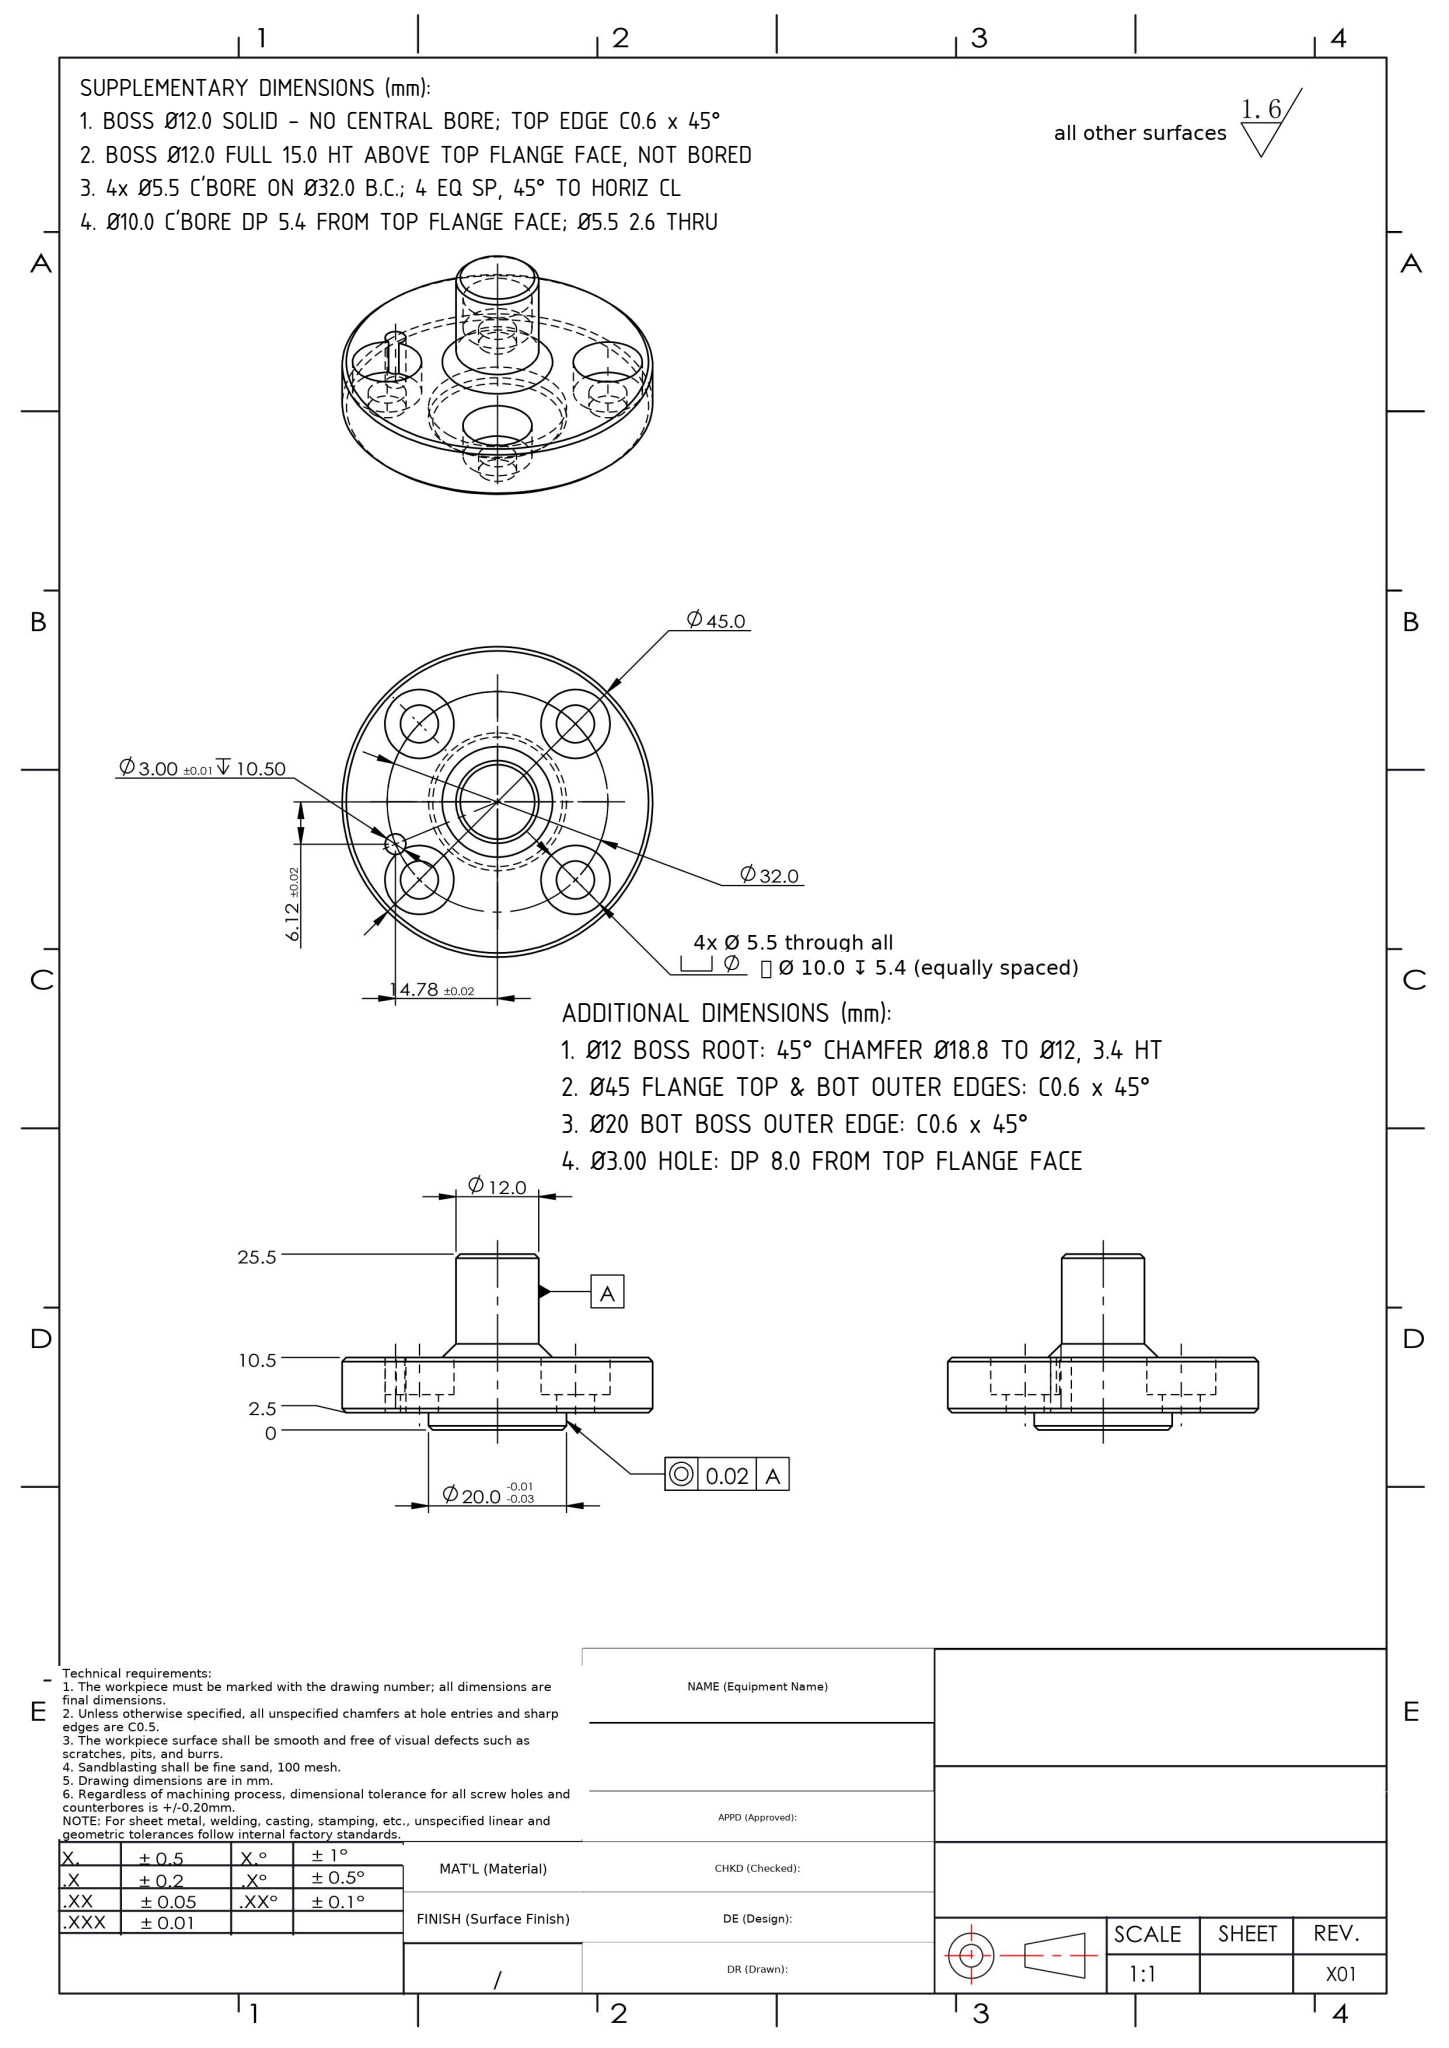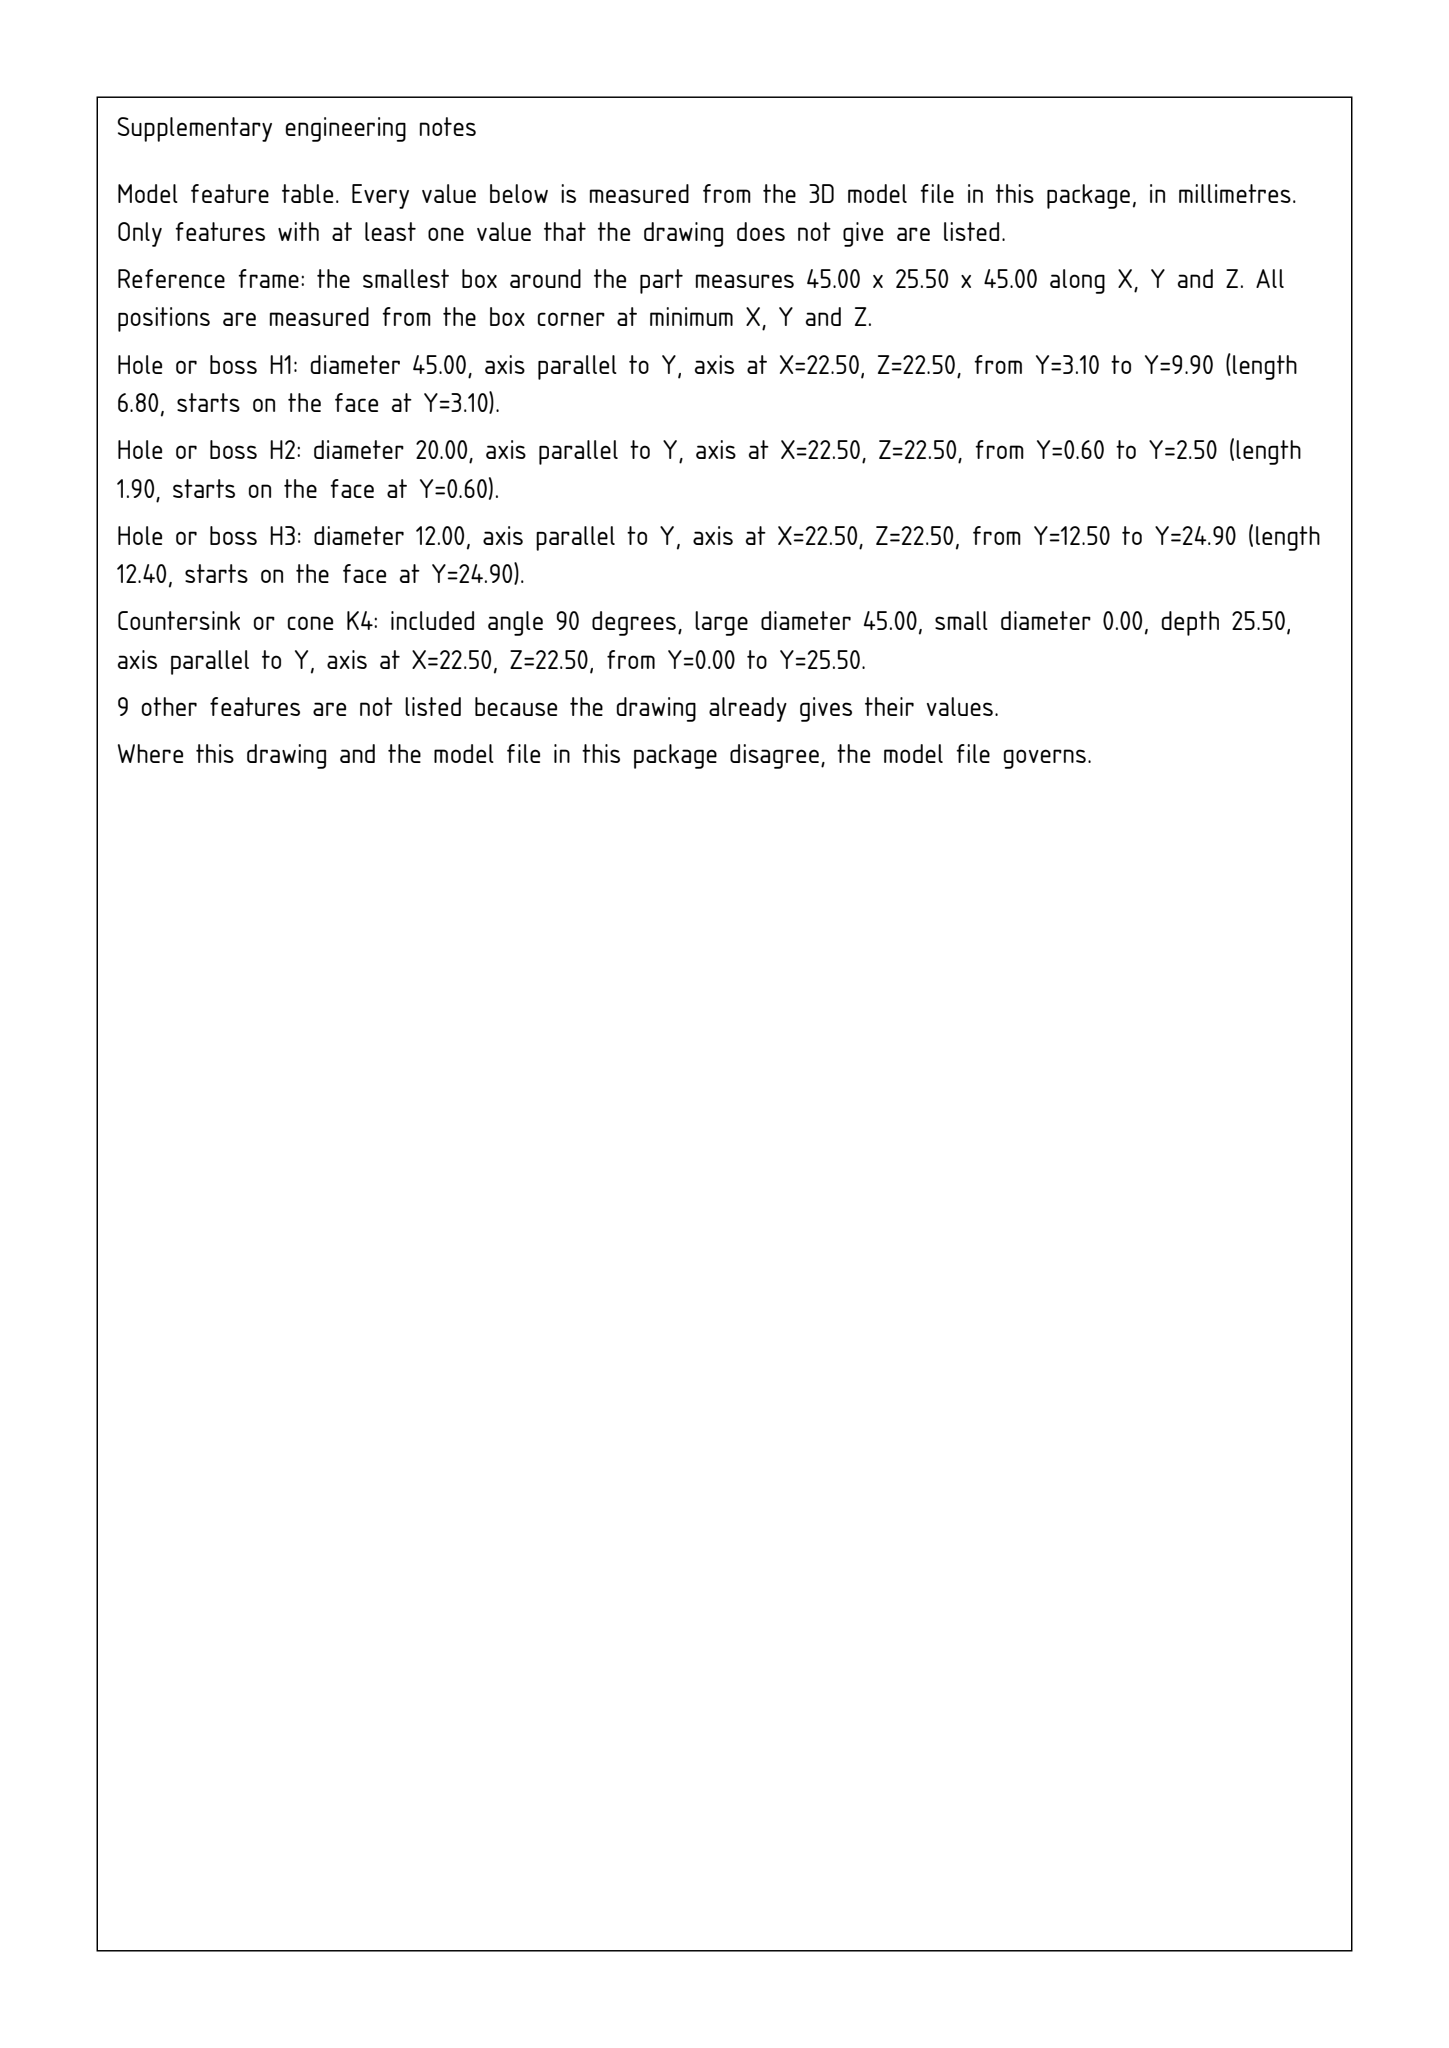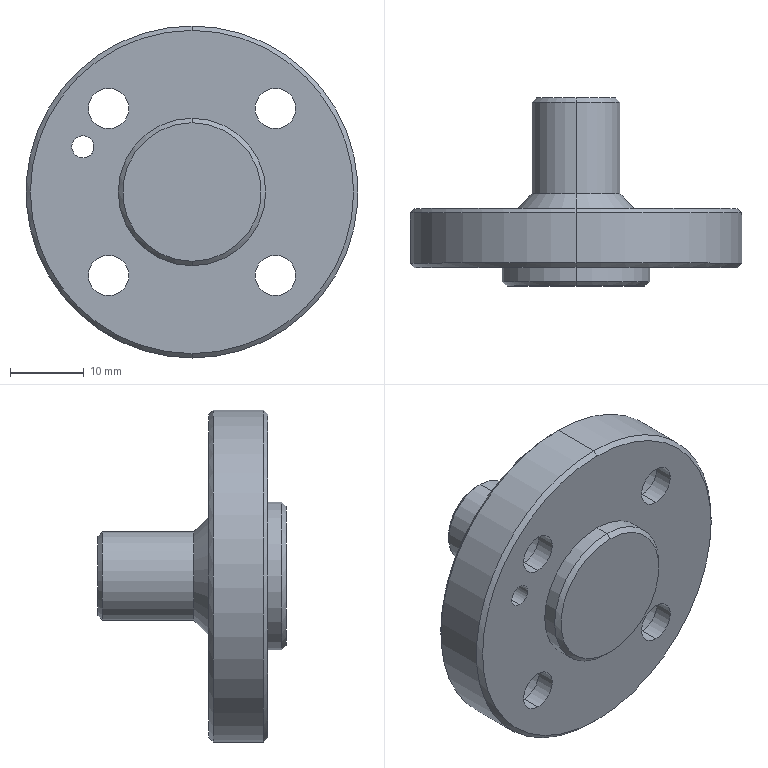Part | SolidWorks | mm | 1 solid | 43 faces | box 45 x 25.5 x 45 mm | volume 13222 mm3 | cylinder 25 | cone 10 | plane 8 | commonest cylinder face diameters 10 x9 5.5 x8 3 x2 20 x2 12 x2 45 x2
build123d program:
from build123d import *

# Parameters (mm, degrees)
SKETCH1_R                                       = 22.5
BOSS_EXTRUDE1_DEPTH                             = 8
SKETCH2_R                                       = 6
BOSS_EXTRUDE2_DEPTH                             = 15
SKETCH3_R                                       = 10
BOSS_EXTRUDE3_DEPTH                             = 2.5
M5_HEX_SOCKET_HEAD_CAP_SCREW_CBORE1_D           = 5.5
M5_HEX_SOCKET_HEAD_CAP_SCREW_CBORE1_CBORE_D     = 10
M5_HEX_SOCKET_HEAD_CAP_SCREW_CBORE1_CBORE_DEPTH = 5.4
CIRPATTERN1_COUNT                               = 4
HOLE1_D                                         = 3
CHAMFER1_SIZE                                   = 0.6
CHAMFER2_SIZE                                   = 2


with BuildPart() as part:
    # Sketch1 → Boss-Extrude1 (new body)
    with BuildSketch(Plane(origin=(0, 0, 0), x_dir=(1, 0, 0), z_dir=(0, 1, 0))):
        with Locations(Location((0, 0, 0), (0, 0, 270))):
            Circle(SKETCH1_R)
    extrude(amount=BOSS_EXTRUDE1_DEPTH)

    # Sketch2 → Boss-Extrude2 (add)
    with BuildSketch(Plane(origin=(0, 8, 0), x_dir=(1, 0, 0), z_dir=(0, 1, 0))):
        with Locations(Location((0, 0, 0), (0, 0, 270))):
            Circle(SKETCH2_R)
    extrude(amount=BOSS_EXTRUDE2_DEPTH)

    # Sketch3 → Boss-Extrude3 (add)
    with BuildSketch(Plane.XZ):
        with Locations(Location((0, 0, 0), (0, 0, 90))):
            Circle(SKETCH3_R)
    extrude(amount=BOSS_EXTRUDE3_DEPTH)

    # M5 Hex Socket Head Cap Screw CBORE1 (through all)
    with Locations(Plane(origin=(0, 8, 0), x_dir=(1, 0, 0), z_dir=(0, 1, 0))):
        with Locations((-11.314, 11.314)):
            m5_hex_socket_head_cap_screw_cbore1 = CounterBoreHole(M5_HEX_SOCKET_HEAD_CAP_SCREW_CBORE1_D / 2, M5_HEX_SOCKET_HEAD_CAP_SCREW_CBORE1_CBORE_D / 2, M5_HEX_SOCKET_HEAD_CAP_SCREW_CBORE1_CBORE_DEPTH)

    # CirPattern1: M5 Hex Socket Head Cap Screw CBORE1 ×4 about axis
    cirpattern1_axis = Axis((0, 0, 0), (0, 1, 0))
    for i in range(1, CIRPATTERN1_COUNT):
        add(m5_hex_socket_head_cap_screw_cbore1.rotate(cirpattern1_axis, i * 360 / CIRPATTERN1_COUNT), mode=Mode.SUBTRACT)

    # Hole1 (through all)
    with Locations(Plane(origin=(0, 8, 0), x_dir=(1, 0, 0), z_dir=(0, 1, 0))):
        with Locations((-14.782, -6.123)):
            Hole(HOLE1_D / 2)

    # Chamfer1
    chamfer1_edges = [part.edges().sort_by_distance(p)[0] for p in [
        (0, -2.5, -10),
        (0, 0, -22.5),
        (0, 8, -22.5),
        (0, 23, -6),
    ]]
    chamfer(chamfer1_edges, length=CHAMFER1_SIZE)

    # Chamfer2
    chamfer2_edges = [part.edges().sort_by_distance(p)[0] for p in [
        (0, 8, -6),
    ]]
    chamfer(chamfer2_edges, length=CHAMFER2_SIZE)


solid = part.part